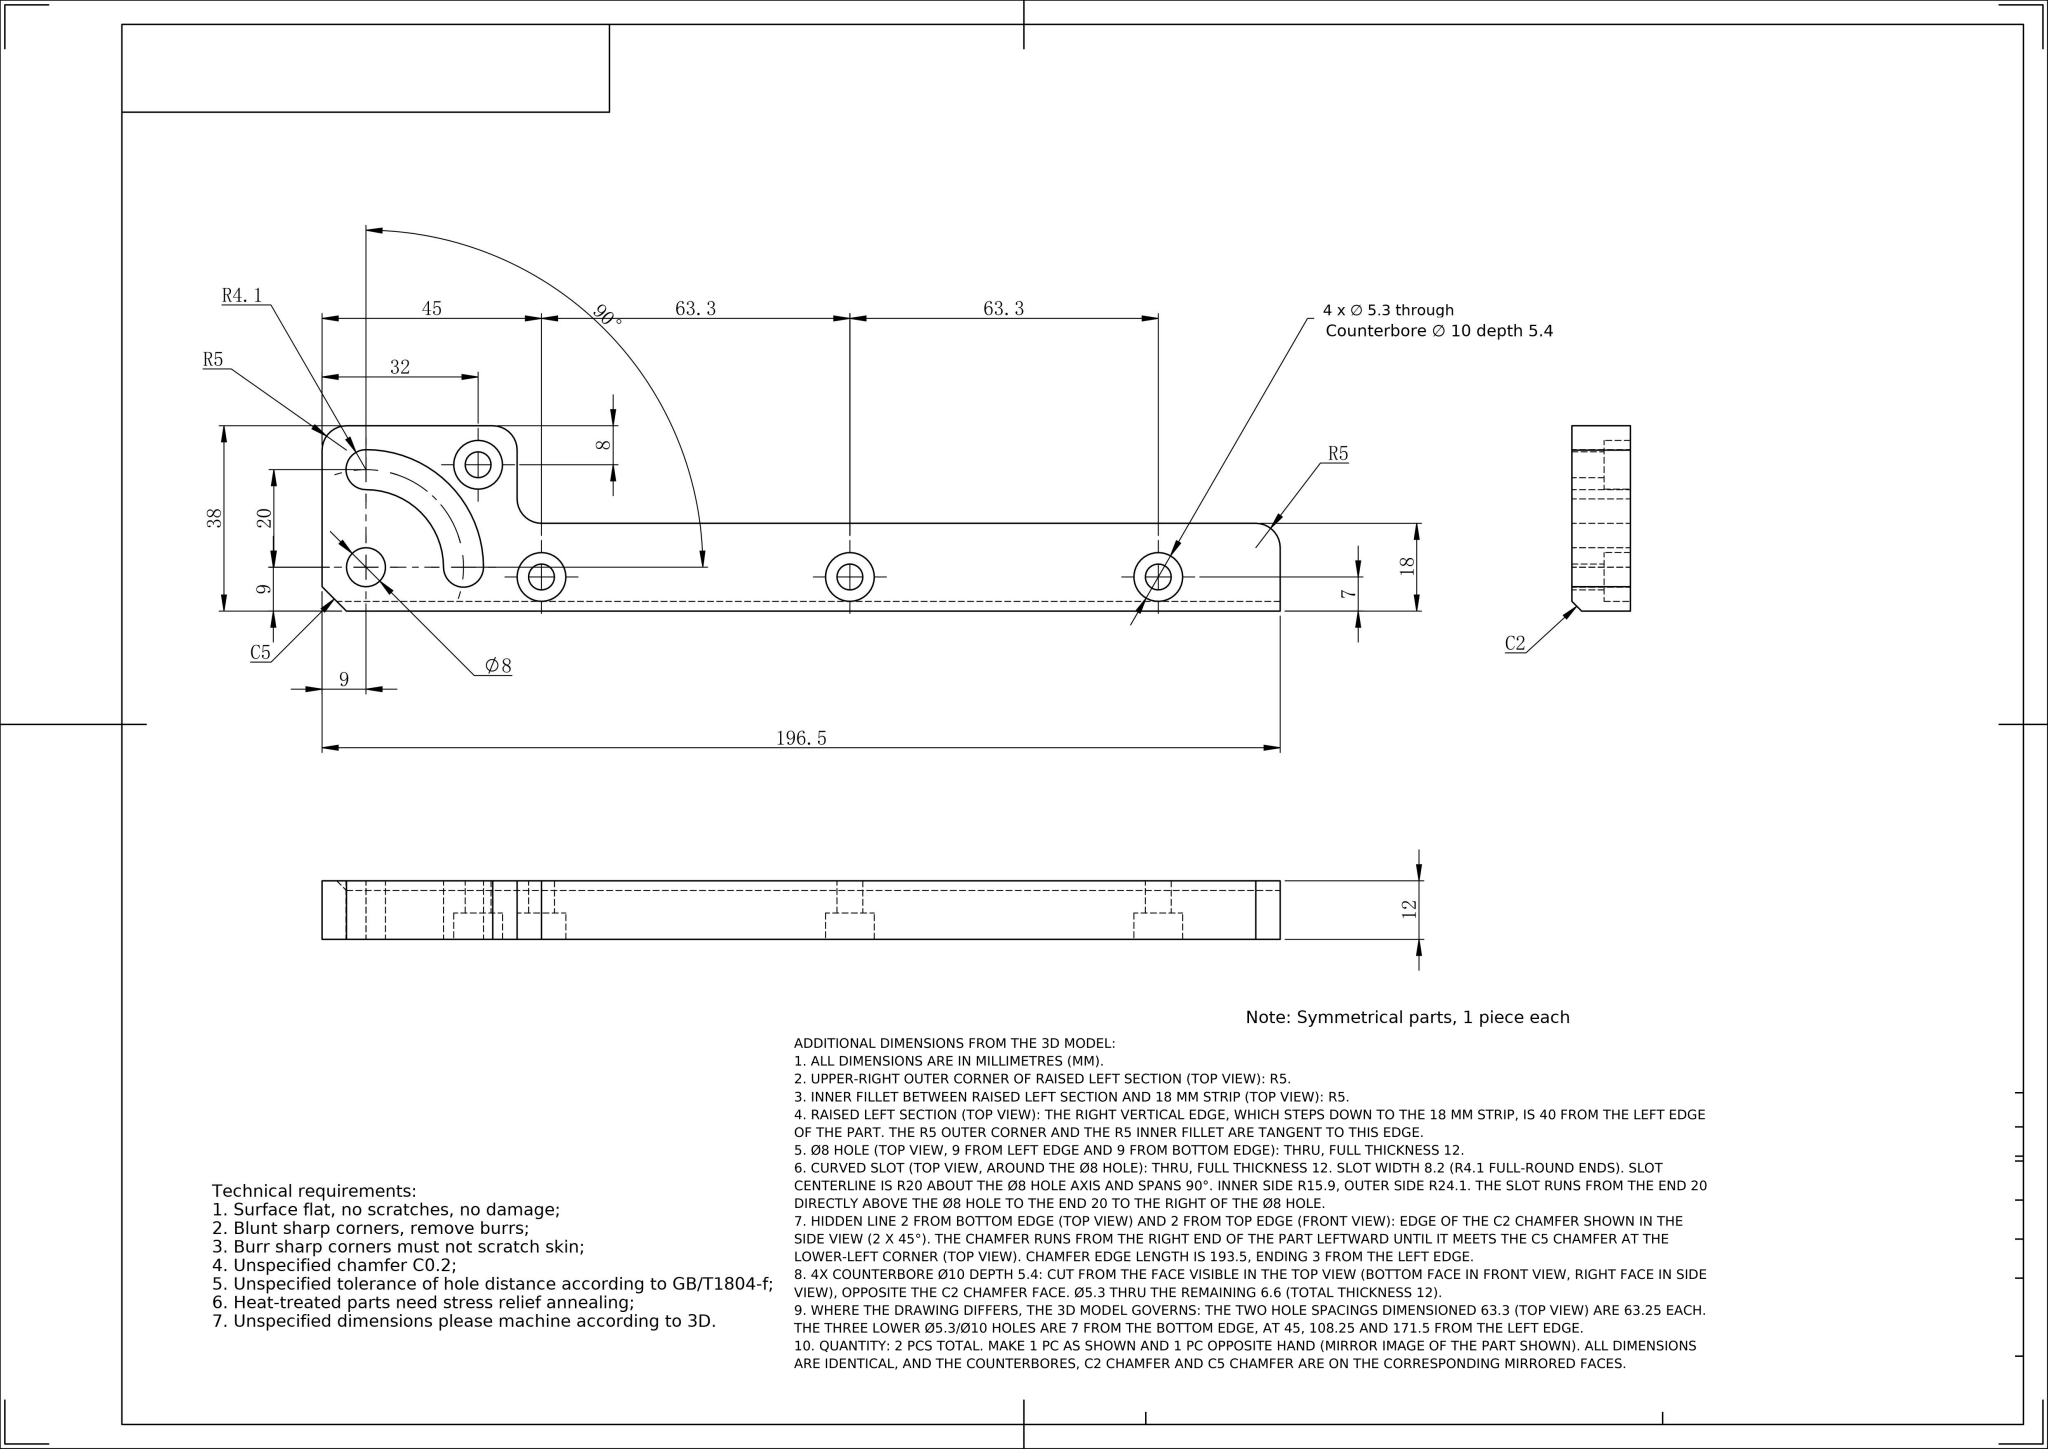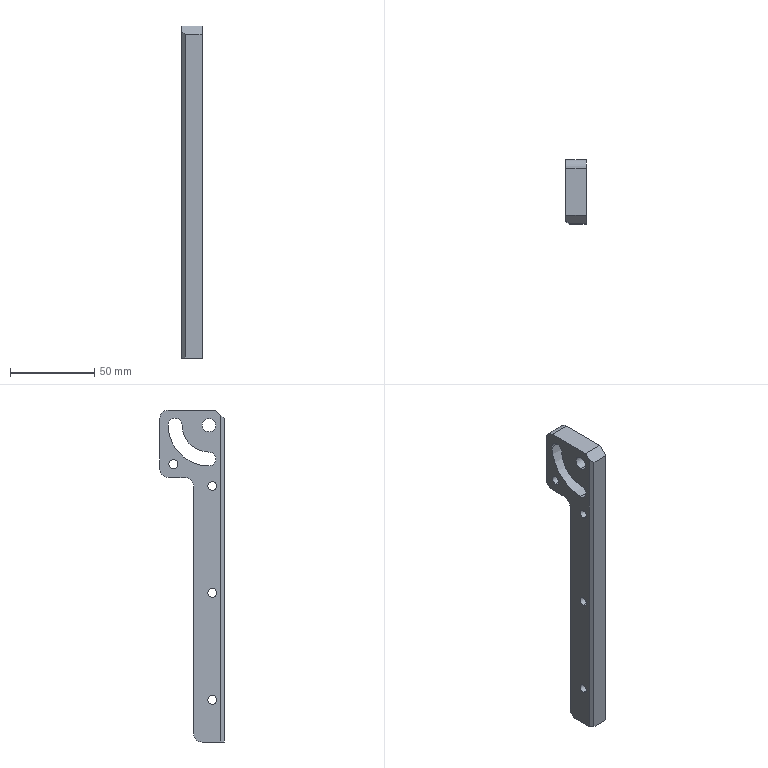Part | NX | mm | 1 solid | 41 faces | box 12 x 38 x 196.5 mm | volume 44774 mm3 | cylinder 27 | plane 14 | commonest cylinder face diameters 10 x12 5.3 x8 8.2 x3 8 x2 31.8 x1 48.2 x1